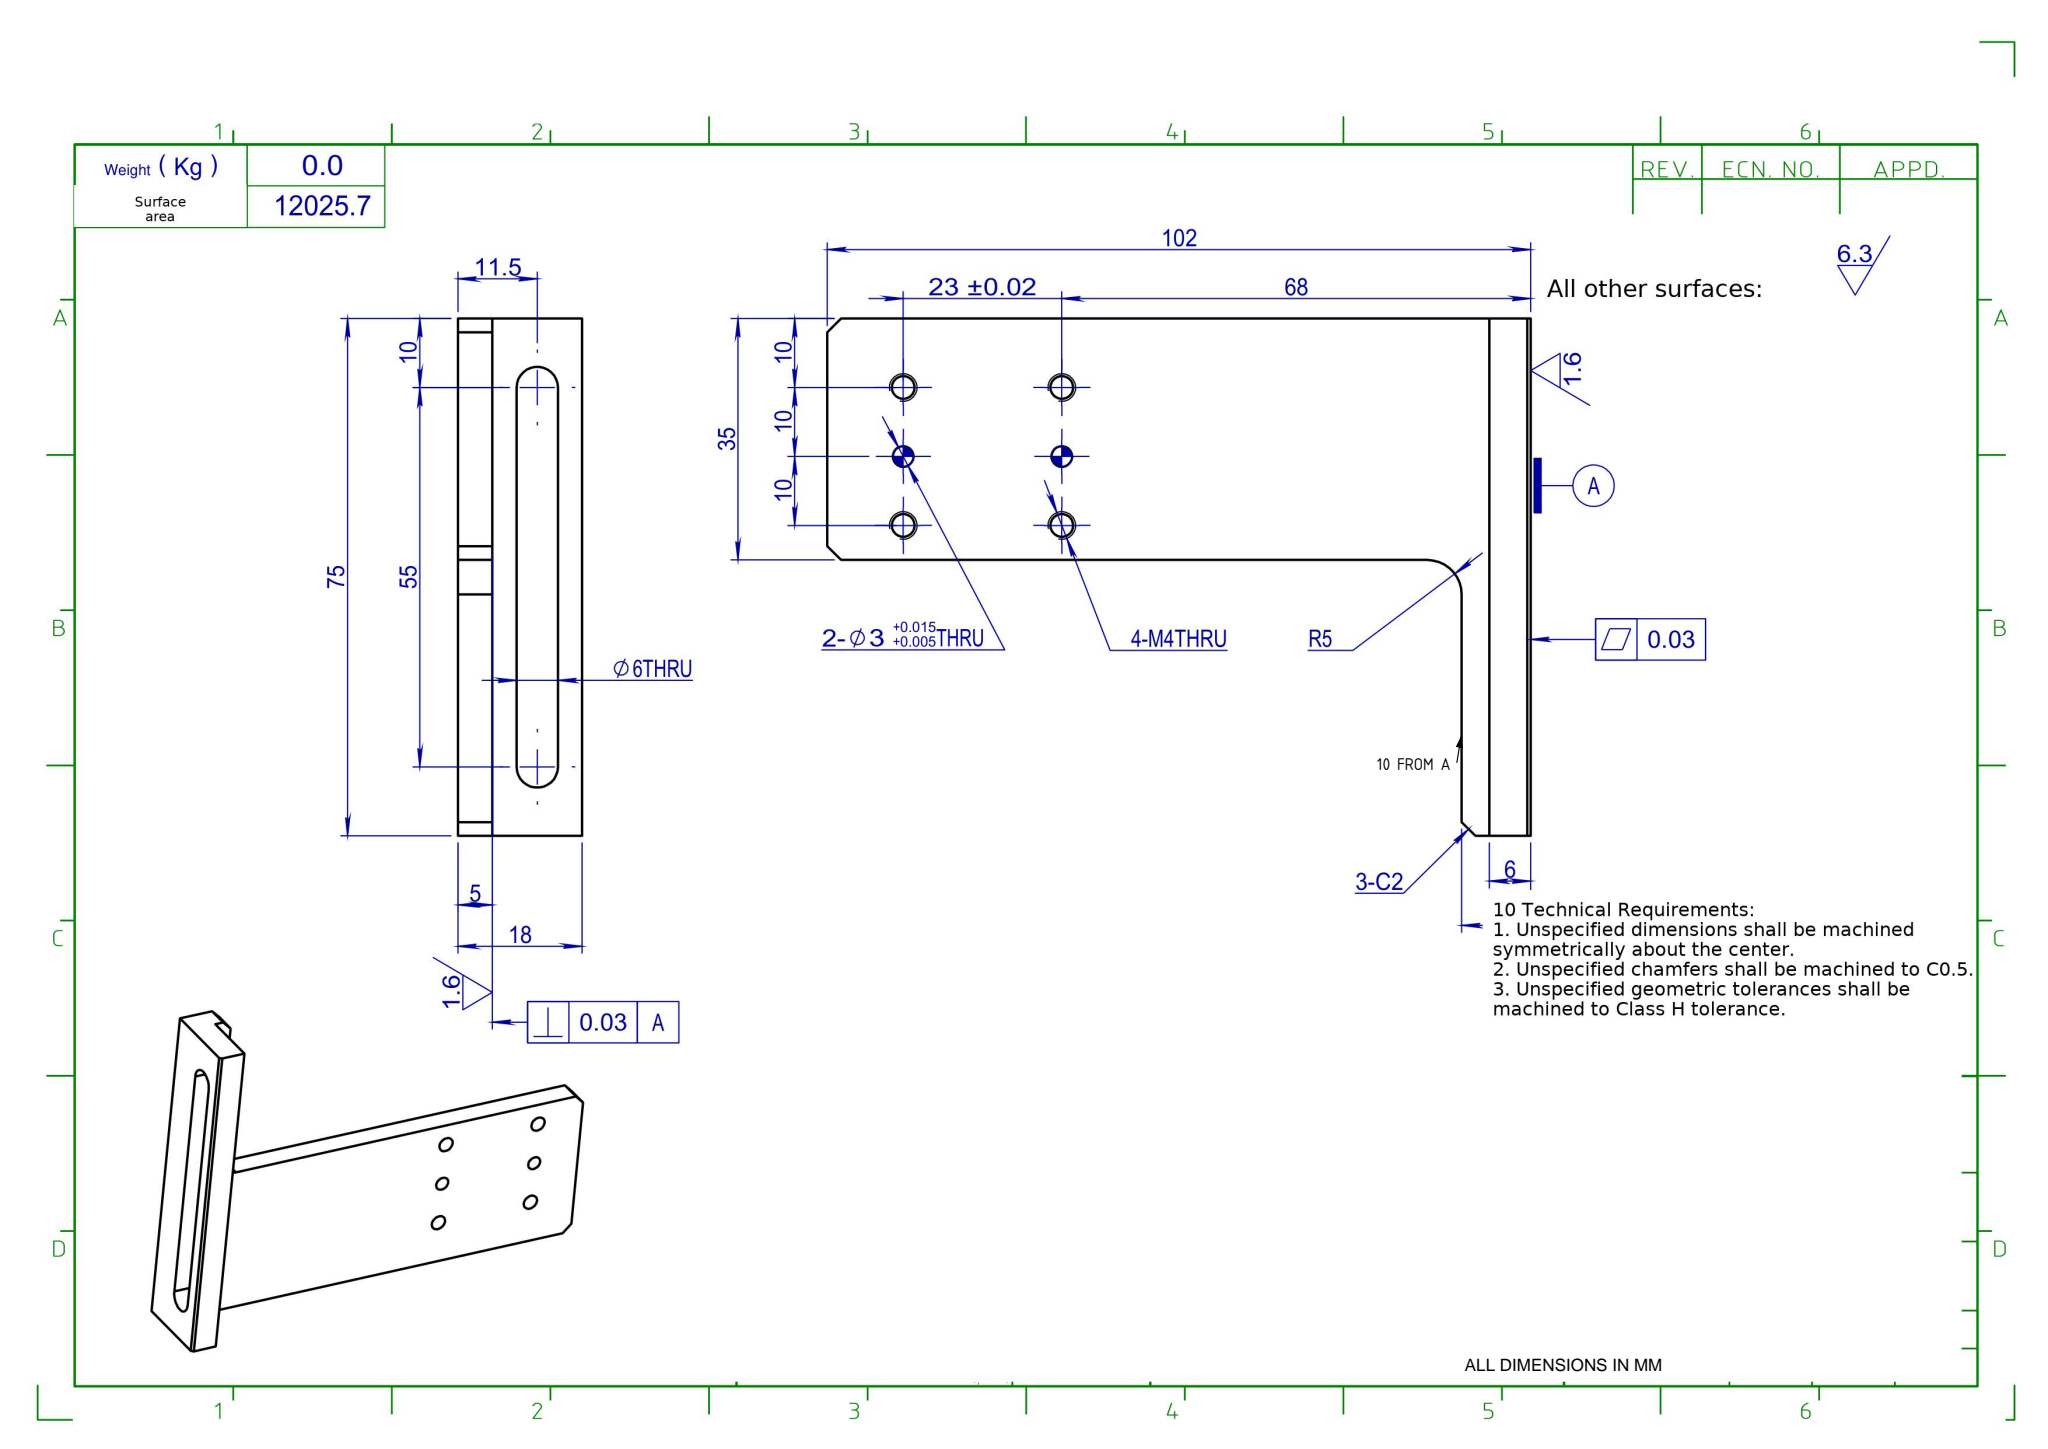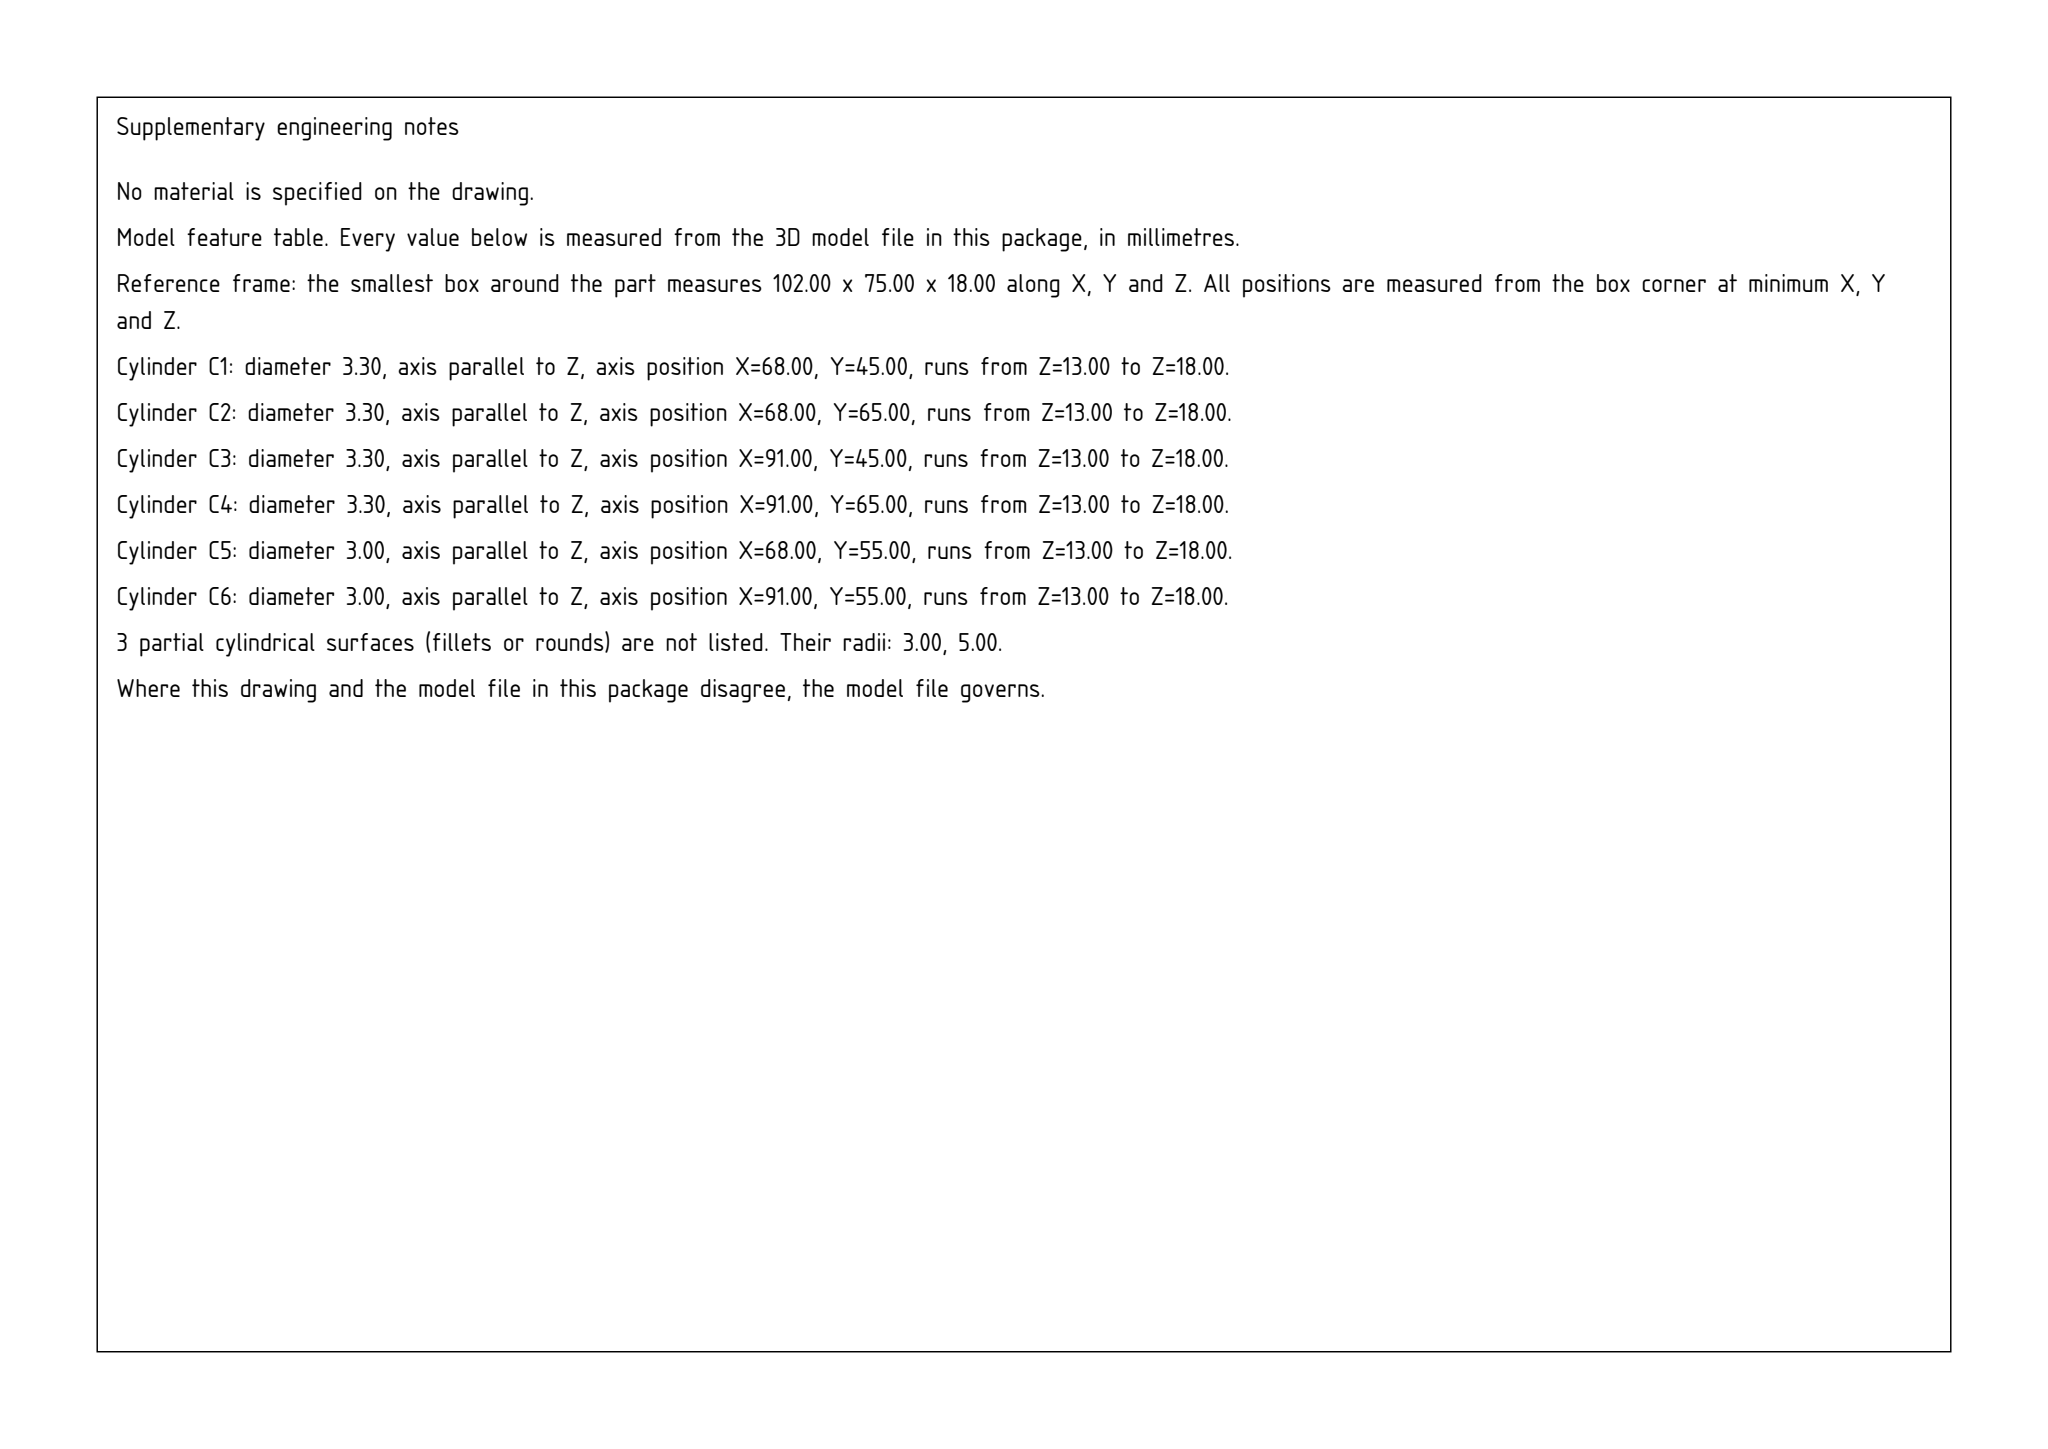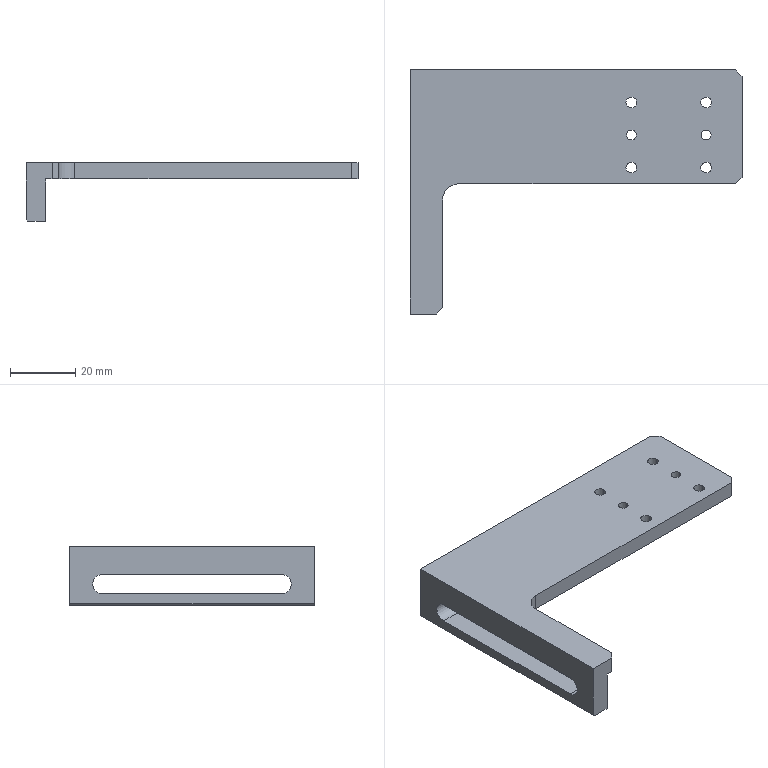Part | SolidWorks | mm | 1 solid | 31 faces | box 102 x 75 x 18 mm | volume 23296 mm3 | plane 16 | cylinder 15 | commonest cylinder face diameters 3.3 x8 3 x4 6 x2 10 x1
Drawing notes:
VERT PLATE STEP: ARM ROOT FACE 10 FROM A (4 ABOVE 6 THK FACE) | from the solid: x-planes at 0 (datum A), 6 (plate back face), 10 (arm root face where R5 is tangent) -> 4 mm step, 10 mm total from A
build123d program:
from build123d import *

# Parameters (mm, degrees)
EXTRUDE1_DEPTH        = 18
FILLET1_R             = 5
CUT_EXTRUDE2_DEPTH    = 149.138
M4_TAPPED_HOLE1_D     = 3.3
M4_TAPPED_HOLE1_DEPTH = 11.5
M4_TAPPED_HOLE1_TIP   = 0.9914
CHAMFER1_SIZE         = 2
SKETCH9_R             = 1.5
CUT_EXTRUDE4_DEPTH    = 112.032
SKETCH10_W            = 92
SKETCH10_H            = 50
CUT_EXTRUDE5_DEPTH    = 13
SKETCH11_W            = 4
SKETCH11_H            = 13
CUT_EXTRUDE6_DEPTH    = 128.879
CHAMFER2_SIZE         = 0.5


with BuildPart() as part:
    # Sketch1 → Extrude1 (new body)
    with BuildSketch(Plane.XY):
        Polygon((-92, 0), (-92, -40), (-102, -40), (-102, 35), (0, 35), (0, 0), align=None)
    extrude(amount=EXTRUDE1_DEPTH)

    # Fillet1
    fillet1_edges = [part.edges().sort_by_distance(p)[0] for p in [
        (-92, 0, 9),
    ]]
    fillet(fillet1_edges, radius=FILLET1_R)

    # Sketch3 → Cut-Extrude2 (cut, through all)
    with BuildSketch(Plane(origin=(-92, 0, -91), x_dir=(0, 0, 1), z_dir=(-1, 0, 0))):
        with BuildLine():
            Line((94.5, 25), (94.5, -30))
            ThreePointArc((94.5, -30), (97.5, -33), (100.5, -30))
            Line((100.5, -30), (100.5, 25))
            ThreePointArc((100.5, 25), (97.5, 28), (94.5, 25))
        make_face()
    extrude(amount=CUT_EXTRUDE2_DEPTH, mode=Mode.SUBTRACT)

    # M4 Tapped Hole1
    with Locations(Plane(origin=(43.908, 9.851, 18), x_dir=(1, 0, 0), z_dir=(0, 0, 1))):
        with Locations((-54.908, -4.851), (-77.908, -4.851), (-77.908, 15.149), (-54.908, 15.149)):
            Hole(M4_TAPPED_HOLE1_D / 2, depth=M4_TAPPED_HOLE1_DEPTH)
            with Locations((0, 0, -(M4_TAPPED_HOLE1_DEPTH + M4_TAPPED_HOLE1_TIP / 2))):  # 118° drill point
                Cone(0, M4_TAPPED_HOLE1_D / 2, M4_TAPPED_HOLE1_TIP, mode=Mode.SUBTRACT)

    # Chamfer1
    chamfer1_edges = [part.edges().sort_by_distance(p)[0] for p in [
        (0, 0, 9),
        (-92, -40, 9),
        (0, 35, 9),
    ]]
    chamfer(chamfer1_edges, length=CHAMFER1_SIZE)

    # Sketch9 → Cut-Extrude4 (cut, through all)
    with BuildSketch(Plane.XY.offset(18)):
        with Locations((-34, 15)):
            Circle(SKETCH9_R)
        with Locations((-11, 15)):
            Circle(SKETCH9_R)
    extrude(amount=-CUT_EXTRUDE4_DEPTH, mode=Mode.SUBTRACT)

    # Sketch10 → Cut-Extrude5 (cut)
    with BuildSketch(Plane(origin=(0, 0, 0), x_dir=(-1, 0, 0), z_dir=(0, 0, -1))):
        with Locations((46, 10)):
            Rectangle(SKETCH10_W, SKETCH10_H)
    extrude(amount=-CUT_EXTRUDE5_DEPTH, mode=Mode.SUBTRACT)

    # Sketch11 → Cut-Extrude6 (cut, through all)
    with BuildSketch(Plane(origin=(0, 35, 0), x_dir=(1, 0, 0), z_dir=(0, 1, 0))):
        with Locations((-94, -6.5)):
            Rectangle(SKETCH11_W, SKETCH11_H)
    extrude(amount=-CUT_EXTRUDE6_DEPTH, mode=Mode.SUBTRACT)

    # Chamfer2
    chamfer2_edges = [part.edges().sort_by_distance(p)[0] for p in [
        (-102, -2.5, 0),
    ]]
    chamfer(chamfer2_edges, length=CHAMFER2_SIZE)


solid = part.part